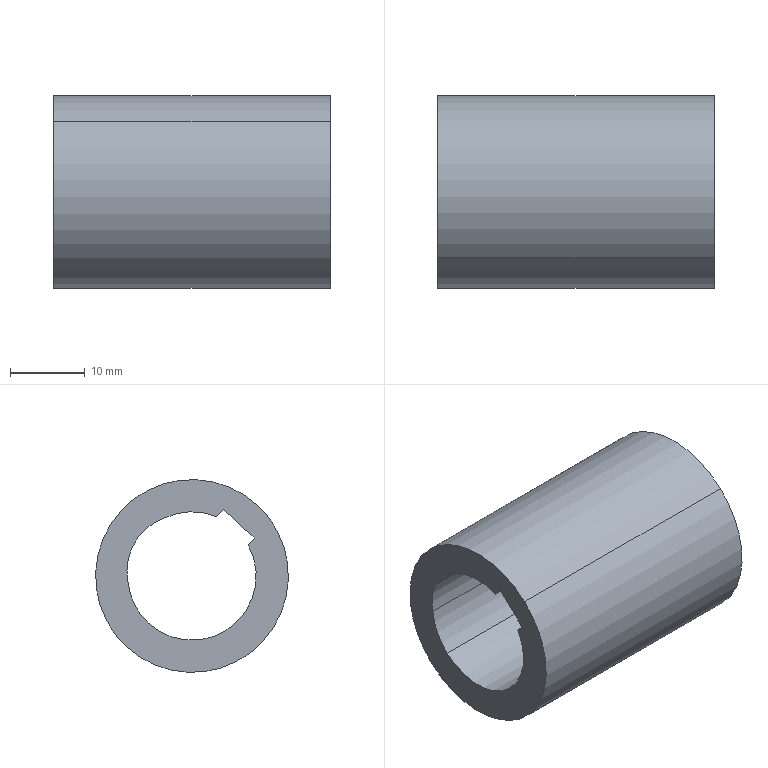Component | SolidWorks | CouplingSleeve-1 | 1 solid | 12 faces | box 37 x 25.76 x 25.76 mm | volume 10448 mm3 | cylinder 6 | plane 6 | commonest cylinder face diameters 17.16 x3 25.756 x2 15 x1
build123d program:
from build123d import *

# Parameters (mm, degrees)
SKETCH2_R                 = 12.878
SKETCH2_R_2               = 8.58
BOSS_EXTRUDE1_DEPTH       = 37
CUT_EXTRUDE1_2_DEPTH      = 66.986
CUT_EXTRUDE1_2_DEPTH_BACK = 66.986
SKETCH1_W                 = 4.594
SKETCH1_H                 = 5.322
CUT_EXTRUDE1_DEPTH        = 66.986


with BuildPart() as part:
    # Sketch2 → Boss-Extrude1 (new body)
    with BuildSketch(Plane(origin=(-166, 0, 0), x_dir=(0, 0, -1), z_dir=(1, 0, 0))):
        with Locations((-40.219, 0)):
            Circle(SKETCH2_R)
        with Locations((-40.219, 0)):
            Circle(SKETCH2_R_2, mode=Mode.SUBTRACT)
    extrude(amount=-BOSS_EXTRUDE1_DEPTH)

    # Sketch4 → Cut-Extrude1_2 (cut, two sides: drawn at the far end of the back side and taken through both)
    with BuildSketch(Plane(origin=(-166, 0, 0), x_dir=(0, 0, -1), z_dir=(1, 0, 0)).offset(-CUT_EXTRUDE1_2_DEPTH_BACK)):
        with BuildLine():
            Line((-46.528, -2.177), (-49.594, -2.177))
            Line((-49.594, -2.177), (-49.594, 3.001))
            Line((-49.594, 3.001), (-47.204, 3.001))
            ThreePointArc((-47.204, 3.001), (-32.458, 2.295), (-46.528, -2.177))
        make_face()
    extrude(amount=CUT_EXTRUDE1_2_DEPTH + CUT_EXTRUDE1_2_DEPTH_BACK, mode=Mode.SUBTRACT)

    # Sketch1 → Cut-Extrude1 (cut, through all)
    with BuildSketch(Plane(origin=(-166, 0, 0), x_dir=(0, 0, -1), z_dir=(1, 0, 0))):
        with Locations((-47.297, 0)):
            Rectangle(SKETCH1_W, SKETCH1_H)
    extrude(amount=-CUT_EXTRUDE1_DEPTH, mode=Mode.SUBTRACT)


solid = part.part

# Placed as in the assembly
solid = solid.moved(Location((-83.5, 87.609, -29.451), (42.923, 0, 0)))
STEP:
#1=COLOUR_RGB('',0.7922,0.8196,0.9333);
#2=FILL_AREA_STYLE_COLOUR('',#1);
#3=FILL_AREA_STYLE('',(#2));
#4=SURFACE_STYLE_FILL_AREA(#3);
#5=SURFACE_SIDE_STYLE('',(#4));
#6=SURFACE_STYLE_USAGE(.BOTH.,#5);
#7=PRESENTATION_STYLE_ASSIGNMENT((#6));
#8=CARTESIAN_POINT('',(-11.28,2.601,-0.2474));
#9=VERTEX_POINT('',#8);
#10=CARTESIAN_POINT('',(-11.28,2.707,-0.03261));
#11=VERTEX_POINT('',#10);
#12=CARTESIAN_POINT('',(-11.28,2.371,-0.));
#13=DIRECTION('',(1.,0.,0.));
#14=DIRECTION('',(0.,0.681,-0.7323));
#15=AXIS2_PLACEMENT_3D('',#12,#13,#14);
#16=CIRCLE('',#15,0.3378);
#17=EDGE_CURVE('',#9,#11,#16,.T.);
#18=ORIENTED_EDGE('',*,*,#17,.F.);
#19=CARTESIAN_POINT('',(-9.823,2.601,-0.2474));
#20=VERTEX_POINT('',#19);
#21=CARTESIAN_POINT('',(-11.28,2.601,-0.2474));
#22=DIRECTION('',(1.,0.,0.));
#23=VECTOR('',#22,39.37);
#24=LINE('',#21,#23);
#25=EDGE_CURVE('',#9,#20,#24,.T.);
#26=ORIENTED_EDGE('',*,*,#25,.T.);
#27=CARTESIAN_POINT('',(-9.823,2.707,-0.03261));
#28=VERTEX_POINT('',#27);
#29=CARTESIAN_POINT('',(-9.823,2.371,-0.));
#30=DIRECTION('',(1.,0.,0.));
#31=DIRECTION('',(0.,0.681,-0.7323));
#32=AXIS2_PLACEMENT_3D('',#29,#30,#31);
#33=CIRCLE('',#32,0.3378);
#34=EDGE_CURVE('',#20,#28,#33,.T.);
#35=ORIENTED_EDGE('',*,*,#34,.T.);
#36=CARTESIAN_POINT('',(-10.551,2.707,-0.03261));
#37=DIRECTION('',(-1.,0.,0.));
#38=VECTOR('',#37,39.37);
#39=LINE('',#36,#38);
#40=EDGE_CURVE('',#28,#11,#39,.T.);
#41=ORIENTED_EDGE('',*,*,#40,.T.);
#42=EDGE_LOOP('',(#18,#26,#35,#41));
#43=FACE_OUTER_BOUND('',#42,.T.);
#44=CARTESIAN_POINT('',(-11.28,2.371,-0.));
#45=DIRECTION('',(1.,0.,0.));
#46=DIRECTION('',(0.,0.681,-0.7323));
#47=AXIS2_PLACEMENT_3D('',#44,#45,#46);
#48=CYLINDRICAL_SURFACE('',#47,0.3378);
#49=ADVANCED_FACE('',(#43),#48,.F.);
#50=CARTESIAN_POINT('',(-11.28,2.716,-0.3713));
#51=VERTEX_POINT('',#50);
#52=CARTESIAN_POINT('',(-11.28,2.026,0.3713));
#53=VERTEX_POINT('',#52);
#54=CARTESIAN_POINT('',(-11.28,2.371,-0.));
#55=DIRECTION('',(1.,0.,0.));
#56=DIRECTION('',(0.,0.681,-0.7323));
#57=AXIS2_PLACEMENT_3D('',#54,#55,#56);
#58=CIRCLE('',#57,0.507);
#59=EDGE_CURVE('',#51,#53,#58,.T.);
#60=ORIENTED_EDGE('',*,*,#59,.T.);
#61=CARTESIAN_POINT('',(-9.823,2.026,0.3713));
#62=VERTEX_POINT('',#61);
#63=CARTESIAN_POINT('',(-11.28,2.026,0.3713));
#64=DIRECTION('',(1.,0.,0.));
#65=VECTOR('',#64,39.37);
#66=LINE('',#63,#65);
#67=EDGE_CURVE('',#53,#62,#66,.T.);
#68=ORIENTED_EDGE('',*,*,#67,.T.);
#69=CARTESIAN_POINT('',(-9.823,2.716,-0.3713));
#70=VERTEX_POINT('',#69);
#71=CARTESIAN_POINT('',(-9.823,2.371,-0.));
#72=DIRECTION('',(1.,0.,0.));
#73=DIRECTION('',(0.,0.681,-0.7323));
#74=AXIS2_PLACEMENT_3D('',#71,#72,#73);
#75=CIRCLE('',#74,0.507);
#76=EDGE_CURVE('',#70,#62,#75,.T.);
#77=ORIENTED_EDGE('',*,*,#76,.F.);
#78=CARTESIAN_POINT('',(-11.28,2.716,-0.3713));
#79=DIRECTION('',(1.,0.,0.));
#80=VECTOR('',#79,39.37);
#81=LINE('',#78,#80);
#82=EDGE_CURVE('',#51,#70,#81,.T.);
#83=ORIENTED_EDGE('',*,*,#82,.F.);
#84=EDGE_LOOP('',(#60,#68,#77,#83));
#85=FACE_OUTER_BOUND('',#84,.T.);
#86=CARTESIAN_POINT('',(-11.28,2.371,-0.));
#87=DIRECTION('',(1.,0.,0.));
#88=DIRECTION('',(0.,0.681,-0.7323));
#89=AXIS2_PLACEMENT_3D('',#86,#87,#88);
#90=CYLINDRICAL_SURFACE('',#89,0.507);
#91=ADVANCED_FACE('',(#85),#90,.T.);
#92=CARTESIAN_POINT('',(-11.28,2.52,0.3031));
#93=VERTEX_POINT('',#92);
#94=CARTESIAN_POINT('',(-11.28,2.242,0.3122));
#95=VERTEX_POINT('',#94);
#96=CARTESIAN_POINT('',(-11.28,2.371,-0.));
#97=DIRECTION('',(1.,0.,0.));
#98=DIRECTION('',(0.,0.681,-0.7323));
#99=AXIS2_PLACEMENT_3D('',#96,#97,#98);
#100=CIRCLE('',#99,0.3378);
#101=EDGE_CURVE('',#93,#95,#100,.T.);
#102=ORIENTED_EDGE('',*,*,#101,.F.);
#103=CARTESIAN_POINT('',(-9.823,2.52,0.3031));
#104=VERTEX_POINT('',#103);
#105=CARTESIAN_POINT('',(-10.551,2.52,0.3031));
#106=DIRECTION('',(1.,0.,0.));
#107=VECTOR('',#106,39.37);
#108=LINE('',#105,#107);
#109=EDGE_CURVE('',#93,#104,#108,.T.);
#110=ORIENTED_EDGE('',*,*,#109,.T.);
#111=CARTESIAN_POINT('',(-9.823,2.242,0.3122));
#112=VERTEX_POINT('',#111);
#113=CARTESIAN_POINT('',(-9.823,2.371,-0.));
#114=DIRECTION('',(1.,0.,0.));
#115=DIRECTION('',(0.,0.681,-0.7323));
#116=AXIS2_PLACEMENT_3D('',#113,#114,#115);
#117=CIRCLE('',#116,0.3378);
#118=EDGE_CURVE('',#104,#112,#117,.T.);
#119=ORIENTED_EDGE('',*,*,#118,.T.);
#120=CARTESIAN_POINT('',(-11.28,2.242,0.3122));
#121=DIRECTION('',(-1.,0.,0.));
#122=VECTOR('',#121,39.37);
#123=LINE('',#120,#122);
#124=EDGE_CURVE('',#112,#95,#123,.T.);
#125=ORIENTED_EDGE('',*,*,#124,.T.);
#126=EDGE_LOOP('',(#102,#110,#119,#125));
#127=FACE_OUTER_BOUND('',#126,.T.);
#128=CARTESIAN_POINT('',(-11.28,2.371,-0.));
#129=DIRECTION('',(1.,0.,0.));
#130=DIRECTION('',(0.,0.681,-0.7323));
#131=AXIS2_PLACEMENT_3D('',#128,#129,#130);
#132=CYLINDRICAL_SURFACE('',#131,0.3378);
#133=ADVANCED_FACE('',(#127),#132,.F.);
#134=ORIENTED_EDGE('',*,*,#67,.F.);
#135=CARTESIAN_POINT('',(-11.28,2.371,-0.));
#136=DIRECTION('',(1.,0.,0.));
#137=DIRECTION('',(0.,0.681,-0.7323));
#138=AXIS2_PLACEMENT_3D('',#135,#136,#137);
#139=CIRCLE('',#138,0.507);
#140=EDGE_CURVE('',#53,#51,#139,.T.);
#141=ORIENTED_EDGE('',*,*,#140,.T.);
#142=ORIENTED_EDGE('',*,*,#82,.T.);
#143=CARTESIAN_POINT('',(-9.823,2.371,-0.));
#144=DIRECTION('',(1.,0.,0.));
#145=DIRECTION('',(0.,0.681,-0.7323));
#146=AXIS2_PLACEMENT_3D('',#143,#144,#145);
#147=CIRCLE('',#146,0.507);
#148=EDGE_CURVE('',#62,#70,#147,.T.);
#149=ORIENTED_EDGE('',*,*,#148,.F.);
#150=EDGE_LOOP('',(#134,#141,#142,#149));
#151=FACE_OUTER_BOUND('',#150,.T.);
#152=CARTESIAN_POINT('',(-11.28,2.371,-0.));
#153=DIRECTION('',(1.,0.,0.));
#154=DIRECTION('',(0.,0.681,-0.7323));
#155=AXIS2_PLACEMENT_3D('',#152,#153,#154);
#156=CYLINDRICAL_SURFACE('',#155,0.507);
#157=ADVANCED_FACE('',(#151),#156,.T.);
#158=CARTESIAN_POINT('',(-11.28,2.057,0.2119));
#159=VERTEX_POINT('',#158);
#160=CARTESIAN_POINT('',(-11.28,2.043,0.1989));
#161=VERTEX_POINT('',#160);
#162=CARTESIAN_POINT('',(-11.28,2.119,0.2703));
#163=DIRECTION('',(0.,-0.7323,-0.681));
#164=VECTOR('',#163,39.37);
#165=LINE('',#162,#164);
#166=EDGE_CURVE('',#159,#161,#165,.T.);
#167=ORIENTED_EDGE('',*,*,#166,.T.);
#168=CARTESIAN_POINT('',(-11.28,2.075,0.1638));
#169=VERTEX_POINT('',#168);
#170=CARTESIAN_POINT('',(-11.28,2.166,0.0665));
#171=DIRECTION('',(0.,0.681,-0.7323));
#172=VECTOR('',#171,39.37);
#173=LINE('',#170,#172);
#174=EDGE_CURVE('',#161,#169,#173,.T.);
#175=ORIENTED_EDGE('',*,*,#174,.T.);
#176=CARTESIAN_POINT('',(-11.28,2.371,-0.));
#177=DIRECTION('',(1.,0.,0.));
#178=DIRECTION('',(0.,0.681,-0.7323));
#179=AXIS2_PLACEMENT_3D('',#176,#177,#178);
#180=CIRCLE('',#179,0.3378);
#181=EDGE_CURVE('',#169,#9,#180,.T.);
#182=ORIENTED_EDGE('',*,*,#181,.T.);
#183=ORIENTED_EDGE('',*,*,#17,.T.);
#184=CARTESIAN_POINT('',(-11.28,2.418,0.02612));
#185=DIRECTION('',(1.,0.,0.));
#186=DIRECTION('',(0.,0.681,-0.7323));
#187=AXIS2_PLACEMENT_3D('',#184,#185,#186);
#188=CIRCLE('',#187,0.2953);
#189=EDGE_CURVE('',#11,#93,#188,.T.);
#190=ORIENTED_EDGE('',*,*,#189,.T.);
#191=ORIENTED_EDGE('',*,*,#101,.T.);
#192=CARTESIAN_POINT('',(-11.28,2.206,0.3507));
#193=VERTEX_POINT('',#192);
#194=CARTESIAN_POINT('',(-11.28,2.206,0.3507));
#195=DIRECTION('',(0.,-0.681,0.7323));
#196=VECTOR('',#195,39.37);
#197=LINE('',#194,#196);
#198=EDGE_CURVE('',#95,#193,#197,.T.);
#199=ORIENTED_EDGE('',*,*,#198,.T.);
#200=CARTESIAN_POINT('',(-11.28,2.119,0.2703));
#201=DIRECTION('',(0.,-0.7323,-0.681));
#202=VECTOR('',#201,39.37);
#203=LINE('',#200,#202);
#204=EDGE_CURVE('',#193,#159,#203,.T.);
#205=ORIENTED_EDGE('',*,*,#204,.T.);
#206=EDGE_LOOP('',(#167,#175,#182,#183,#190,#191,#199,#205));
#207=FACE_BOUND('',#206,.T.);
#208=ORIENTED_EDGE('',*,*,#59,.F.);
#209=ORIENTED_EDGE('',*,*,#140,.F.);
#210=EDGE_LOOP('',(#208,#209));
#211=FACE_OUTER_BOUND('',#210,.T.);
#212=CARTESIAN_POINT('',(-11.28,2.371,-0.));
#213=DIRECTION('',(1.,0.,0.));
#214=DIRECTION('',(0.,0.681,-0.7323));
#215=AXIS2_PLACEMENT_3D('',#212,#213,#214);
#216=PLANE('',#215);
#217=ADVANCED_FACE('',(#207,#211),#216,.F.);
#218=CARTESIAN_POINT('',(-9.823,2.057,0.2119));
#219=VERTEX_POINT('',#218);
#220=CARTESIAN_POINT('',(-9.823,2.043,0.1989));
#221=VERTEX_POINT('',#220);
#222=CARTESIAN_POINT('',(-9.823,2.043,0.1989));
#223=DIRECTION('',(0.,-0.7323,-0.681));
#224=VECTOR('',#223,39.37);
#225=LINE('',#222,#224);
#226=EDGE_CURVE('',#219,#221,#225,.T.);
#227=ORIENTED_EDGE('',*,*,#226,.F.);
#228=CARTESIAN_POINT('',(-9.823,2.206,0.3507));
#229=VERTEX_POINT('',#228);
#230=CARTESIAN_POINT('',(-9.823,2.057,0.2119));
#231=DIRECTION('',(0.,-0.7323,-0.681));
#232=VECTOR('',#231,39.37);
#233=LINE('',#230,#232);
#234=EDGE_CURVE('',#229,#219,#233,.T.);
#235=ORIENTED_EDGE('',*,*,#234,.F.);
#236=CARTESIAN_POINT('',(-9.823,2.457,0.08045));
#237=DIRECTION('',(0.,-0.681,0.7323));
#238=VECTOR('',#237,39.37);
#239=LINE('',#236,#238);
#240=EDGE_CURVE('',#112,#229,#239,.T.);
#241=ORIENTED_EDGE('',*,*,#240,.F.);
#242=ORIENTED_EDGE('',*,*,#118,.F.);
#243=CARTESIAN_POINT('',(-9.823,2.418,0.02612));
#244=DIRECTION('',(1.,0.,0.));
#245=DIRECTION('',(0.,0.681,-0.7323));
#246=AXIS2_PLACEMENT_3D('',#243,#244,#245);
#247=CIRCLE('',#246,0.2953);
#248=EDGE_CURVE('',#28,#104,#247,.T.);
#249=ORIENTED_EDGE('',*,*,#248,.F.);
#250=ORIENTED_EDGE('',*,*,#34,.F.);
#251=CARTESIAN_POINT('',(-9.823,2.075,0.1638));
#252=VERTEX_POINT('',#251);
#253=CARTESIAN_POINT('',(-9.823,2.371,-0.));
#254=DIRECTION('',(1.,0.,0.));
#255=DIRECTION('',(0.,0.681,-0.7323));
#256=AXIS2_PLACEMENT_3D('',#253,#254,#255);
#257=CIRCLE('',#256,0.3378);
#258=EDGE_CURVE('',#252,#20,#257,.T.);
#259=ORIENTED_EDGE('',*,*,#258,.F.);
#260=CARTESIAN_POINT('',(-9.823,2.166,0.0665));
#261=DIRECTION('',(0.,0.681,-0.7323));
#262=VECTOR('',#261,39.37);
#263=LINE('',#260,#262);
#264=EDGE_CURVE('',#221,#252,#263,.T.);
#265=ORIENTED_EDGE('',*,*,#264,.F.);
#266=EDGE_LOOP('',(#227,#235,#241,#242,#249,#250,#259,#265));
#267=FACE_BOUND('',#266,.T.);
#268=ORIENTED_EDGE('',*,*,#76,.T.);
#269=ORIENTED_EDGE('',*,*,#148,.T.);
#270=EDGE_LOOP('',(#268,#269));
#271=FACE_OUTER_BOUND('',#270,.T.);
#272=CARTESIAN_POINT('',(-9.823,2.371,-0.));
#273=DIRECTION('',(1.,0.,0.));
#274=DIRECTION('',(0.,0.681,-0.7323));
#275=AXIS2_PLACEMENT_3D('',#272,#273,#274);
#276=PLANE('',#275);
#277=ADVANCED_FACE('',(#267,#271),#276,.T.);
#278=ORIENTED_EDGE('',*,*,#25,.F.);
#279=ORIENTED_EDGE('',*,*,#181,.F.);
#280=CARTESIAN_POINT('',(-11.28,2.075,0.1638));
#281=DIRECTION('',(1.,0.,0.));
#282=VECTOR('',#281,39.37);
#283=LINE('',#280,#282);
#284=EDGE_CURVE('',#169,#252,#283,.T.);
#285=ORIENTED_EDGE('',*,*,#284,.T.);
#286=ORIENTED_EDGE('',*,*,#258,.T.);
#287=EDGE_LOOP('',(#278,#279,#285,#286));
#288=FACE_OUTER_BOUND('',#287,.T.);
#289=CARTESIAN_POINT('',(-11.28,2.371,-0.));
#290=DIRECTION('',(1.,0.,0.));
#291=DIRECTION('',(0.,0.681,-0.7323));
#292=AXIS2_PLACEMENT_3D('',#289,#290,#291);
#293=CYLINDRICAL_SURFACE('',#292,0.3378);
#294=ADVANCED_FACE('',(#288),#293,.F.);
#295=ORIENTED_EDGE('',*,*,#240,.T.);
#296=CARTESIAN_POINT('',(-11.28,2.206,0.3507));
#297=DIRECTION('',(1.,0.,0.));
#298=VECTOR('',#297,39.37);
#299=LINE('',#296,#298);
#300=EDGE_CURVE('',#193,#229,#299,.T.);
#301=ORIENTED_EDGE('',*,*,#300,.F.);
#302=ORIENTED_EDGE('',*,*,#198,.F.);
#303=ORIENTED_EDGE('',*,*,#124,.F.);
#304=EDGE_LOOP('',(#295,#301,#302,#303));
#305=FACE_OUTER_BOUND('',#304,.T.);
#306=CARTESIAN_POINT('',(-11.28,2.206,0.3507));
#307=DIRECTION('',(0.,0.7323,0.681));
#308=DIRECTION('',(0.,-0.681,0.7323));
#309=AXIS2_PLACEMENT_3D('',#306,#307,#308);
#310=PLANE('',#309);
#311=ADVANCED_FACE('',(#305),#310,.F.);
#312=CARTESIAN_POINT('',(-11.28,2.057,0.2119));
#313=CARTESIAN_POINT('',(-10.794,2.057,0.2119));
#314=CARTESIAN_POINT('',(-10.308,2.057,0.2119));
#315=CARTESIAN_POINT('',(-9.823,2.057,0.2119));
#316=B_SPLINE_CURVE_WITH_KNOTS('',3,(#312,#313,#314,#315),.UNSPECIFIED.,.F.,.F.,(4,4),(0.,1.),.UNSPECIFIED.);
#317=EDGE_CURVE('',#159,#219,#316,.T.);
#318=ORIENTED_EDGE('',*,*,#317,.F.);
#319=ORIENTED_EDGE('',*,*,#204,.F.);
#320=ORIENTED_EDGE('',*,*,#300,.T.);
#321=ORIENTED_EDGE('',*,*,#234,.T.);
#322=EDGE_LOOP('',(#318,#319,#320,#321));
#323=FACE_OUTER_BOUND('',#322,.T.);
#324=CARTESIAN_POINT('',(-11.28,2.057,0.2119));
#325=DIRECTION('',(0.,-0.681,0.7323));
#326=DIRECTION('',(1.,0.,0.));
#327=AXIS2_PLACEMENT_3D('',#324,#325,#326);
#328=PLANE('',#327);
#329=ADVANCED_FACE('',(#323),#328,.F.);
#330=ORIENTED_EDGE('',*,*,#189,.F.);
#331=ORIENTED_EDGE('',*,*,#40,.F.);
#332=ORIENTED_EDGE('',*,*,#248,.T.);
#333=ORIENTED_EDGE('',*,*,#109,.F.);
#334=EDGE_LOOP('',(#330,#331,#332,#333));
#335=FACE_OUTER_BOUND('',#334,.T.);
#336=CARTESIAN_POINT('',(-11.28,2.418,0.02612));
#337=DIRECTION('',(1.,0.,0.));
#338=DIRECTION('',(0.,0.681,-0.7323));
#339=AXIS2_PLACEMENT_3D('',#336,#337,#338);
#340=CYLINDRICAL_SURFACE('',#339,0.2953);
#341=ADVANCED_FACE('',(#335),#340,.F.);
#342=ORIENTED_EDGE('',*,*,#174,.F.);
#343=CARTESIAN_POINT('',(-11.28,2.043,0.1989));
#344=DIRECTION('',(1.,0.,0.));
#345=VECTOR('',#344,39.37);
#346=LINE('',#343,#345);
#347=EDGE_CURVE('',#161,#221,#346,.T.);
#348=ORIENTED_EDGE('',*,*,#347,.T.);
#349=ORIENTED_EDGE('',*,*,#264,.T.);
#350=ORIENTED_EDGE('',*,*,#284,.F.);
#351=EDGE_LOOP('',(#342,#348,#349,#350));
#352=FACE_OUTER_BOUND('',#351,.T.);
#353=CARTESIAN_POINT('',(-11.28,2.166,0.0665));
#354=DIRECTION('',(0.,-0.7323,-0.681));
#355=DIRECTION('',(0.,0.681,-0.7323));
#356=AXIS2_PLACEMENT_3D('',#353,#354,#355);
#357=PLANE('',#356);
#358=ADVANCED_FACE('',(#352),#357,.F.);
#359=ORIENTED_EDGE('',*,*,#317,.T.);
#360=ORIENTED_EDGE('',*,*,#226,.T.);
#361=ORIENTED_EDGE('',*,*,#347,.F.);
#362=ORIENTED_EDGE('',*,*,#166,.F.);
#363=EDGE_LOOP('',(#359,#360,#361,#362));
#364=FACE_OUTER_BOUND('',#363,.T.);
#365=CARTESIAN_POINT('',(-11.28,2.043,0.1989));
#366=DIRECTION('',(0.,-0.681,0.7323));
#367=DIRECTION('',(1.,0.,0.));
#368=AXIS2_PLACEMENT_3D('',#365,#366,#367);
#369=PLANE('',#368);
#370=ADVANCED_FACE('',(#364),#369,.F.);
#371=CLOSED_SHELL('',(#49,#91,#133,#157,#217,#277,#294,#311,#329,#341,#358,#370));
#372=MANIFOLD_SOLID_BREP('',#371);
#373=STYLED_ITEM('',(#7),#372);
#374=(LENGTH_UNIT()NAMED_UNIT(*)SI_UNIT($,.METRE.));
#375=LENGTH_MEASURE_WITH_UNIT(LENGTH_MEASURE(0.0254),#374);
#376=DIMENSIONAL_EXPONENTS(1.,0.,0.,0.,0.,0.,0.);
#377=(CONVERSION_BASED_UNIT('',#375)LENGTH_UNIT()NAMED_UNIT(#376));
#378=UNCERTAINTY_MEASURE_WITH_UNIT(LENGTH_MEASURE(0.00001),#377,'','');
#379=(NAMED_UNIT(*)PLANE_ANGLE_UNIT()SI_UNIT($,.RADIAN.));
#380=(NAMED_UNIT(*)SI_UNIT($,.STERADIAN.)SOLID_ANGLE_UNIT());
#381=(GEOMETRIC_REPRESENTATION_CONTEXT(3)GLOBAL_UNCERTAINTY_ASSIGNED_CONTEXT((#378))GLOBAL_UNIT_ASSIGNED_CONTEXT((#377,#379,#380))REPRESENTATION_CONTEXT('',''));
#382=MECHANICAL_DESIGN_GEOMETRIC_PRESENTATION_REPRESENTATION('',(#373),#381);
#383=CARTESIAN_POINT('',(0.,0.,0.));
#384=DIRECTION('',(0.,0.,1.));
#385=DIRECTION('',(1.,0.,0.));
#386=AXIS2_PLACEMENT_3D('',#383,#384,#385);
#387=(LENGTH_UNIT()NAMED_UNIT(*)SI_UNIT($,.METRE.));
#388=LENGTH_MEASURE_WITH_UNIT(LENGTH_MEASURE(0.0254),#387);
#389=DIMENSIONAL_EXPONENTS(1.,0.,0.,0.,0.,0.,0.);
#390=(CONVERSION_BASED_UNIT('',#388)LENGTH_UNIT()NAMED_UNIT(#389));
#391=UNCERTAINTY_MEASURE_WITH_UNIT(LENGTH_MEASURE(0.00001),#390,'','');
#392=(NAMED_UNIT(*)PLANE_ANGLE_UNIT()SI_UNIT($,.RADIAN.));
#393=(NAMED_UNIT(*)SI_UNIT($,.STERADIAN.)SOLID_ANGLE_UNIT());
#394=(GEOMETRIC_REPRESENTATION_CONTEXT(3)GLOBAL_UNCERTAINTY_ASSIGNED_CONTEXT((#391))GLOBAL_UNIT_ASSIGNED_CONTEXT((#390,#392,#393))REPRESENTATION_CONTEXT('',''));
#395=ADVANCED_BREP_SHAPE_REPRESENTATION('',(#372,#386),#394);
#396=PRESENTATION_LAYER_ASSIGNMENT('','',(#373));